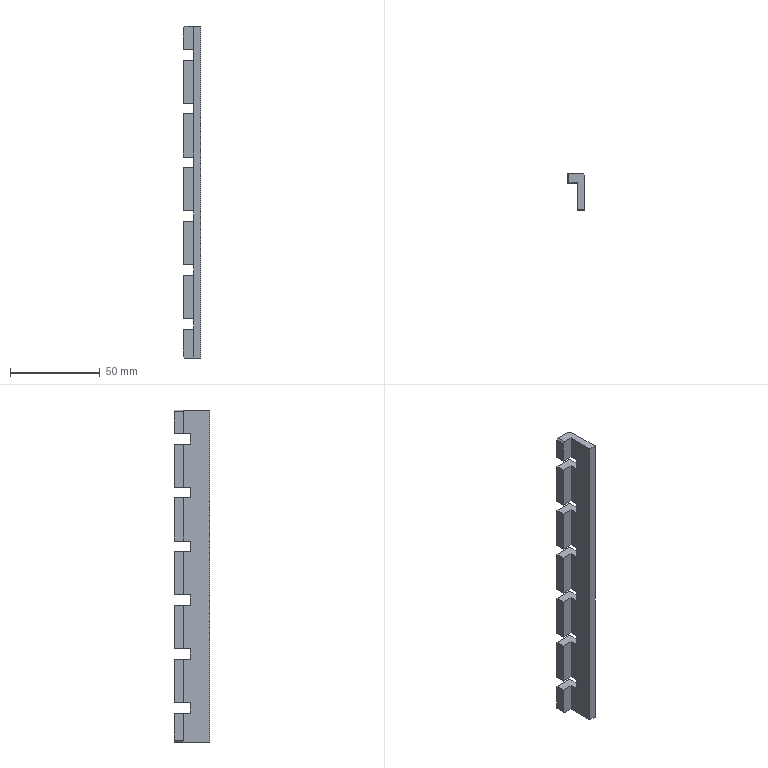Component | SolidWorks | Inline-H010-H01160308-006K-1 | 1 solid | 53 faces | box 10 x 20 x 185 mm | volume 17977 mm3 | plane 53
build123d program:
from build123d import *

# Parameters (mm, degrees)
SKETCH1_W           = 20
SKETCH1_H           = 10
BOSS_EXTRUDE1_DEPTH = 92.5
SKETCH2_W           = 14.899
SKETCH2_H           = 6
CUT_EXTRUDE1_DEPTH  = 196.712
SKETCH3_W           = 9.052
SKETCH3_H           = 6
CUT_EXTRUDE2_DEPTH  = 96.164
LPATTERN1_COUNT     = 6
LPATTERN1_PITCH     = 30
CHAMFER1_SIZE       = 1
CHAMFER2_SIZE       = 1


with BuildPart() as part:
    # Sketch1 → Boss-Extrude1 (new, symmetric)
    with BuildSketch(Plane.XY):
        with Locations((10, 55.648)):
            Rectangle(SKETCH1_W, SKETCH1_H)
    extrude(amount=BOSS_EXTRUDE1_DEPTH, both=True)

    # Sketch2 → Cut-Extrude1 (cut, through all)
    with BuildSketch(Plane.XY.offset(92.5)):
        with Locations((12.551, 53.648)):
            Rectangle(SKETCH2_W, SKETCH2_H)
    extrude(amount=-CUT_EXTRUDE1_DEPTH, mode=Mode.SUBTRACT)

    # Sketch3 → Cut-Extrude2 (cut, through all)
    with BuildSketch(Plane(origin=(0, 60.648, 0), x_dir=(1, 0, 0), z_dir=(0, 1, 0))):
        with Locations((4.526, -76.5)):
            Rectangle(SKETCH3_W, SKETCH3_H)
    cut_extrude2 = extrude(amount=-CUT_EXTRUDE2_DEPTH, mode=Mode.SUBTRACT)

    # LPattern1: Cut-Extrude2 ×6
    with Locations(*[(0, 0, -i * LPATTERN1_PITCH) for i in range(1, LPATTERN1_COUNT)]):
        add(cut_extrude2, mode=Mode.SUBTRACT)

    # Chamfer1
    chamfer1_edges = [part.edges().sort_by_distance(p)[0] for p in [
        (2.551, 50.648, 92.5),
        (2.551, 50.648, -92.5),
    ]]
    chamfer(chamfer1_edges, length=CHAMFER1_SIZE)

    # Chamfer2
    chamfer2_edges = [part.edges().sort_by_distance(p)[0] for p in [
        (0, 60.648, -58.5),
        (0, 60.648, -84.5),
        (0, 60.648, 61.5),
        (0, 60.648, 31.5),
        (0, 60.648, 1.5),
        (0, 60.648, 86),
        (0, 60.648, -28.5),
    ]]
    chamfer(chamfer2_edges, length=CHAMFER2_SIZE)


solid = part.part

# Placed as in the assembly
solid = solid.moved(Location((-6.88, 51.968, 139.665), (0, 0, -90)))